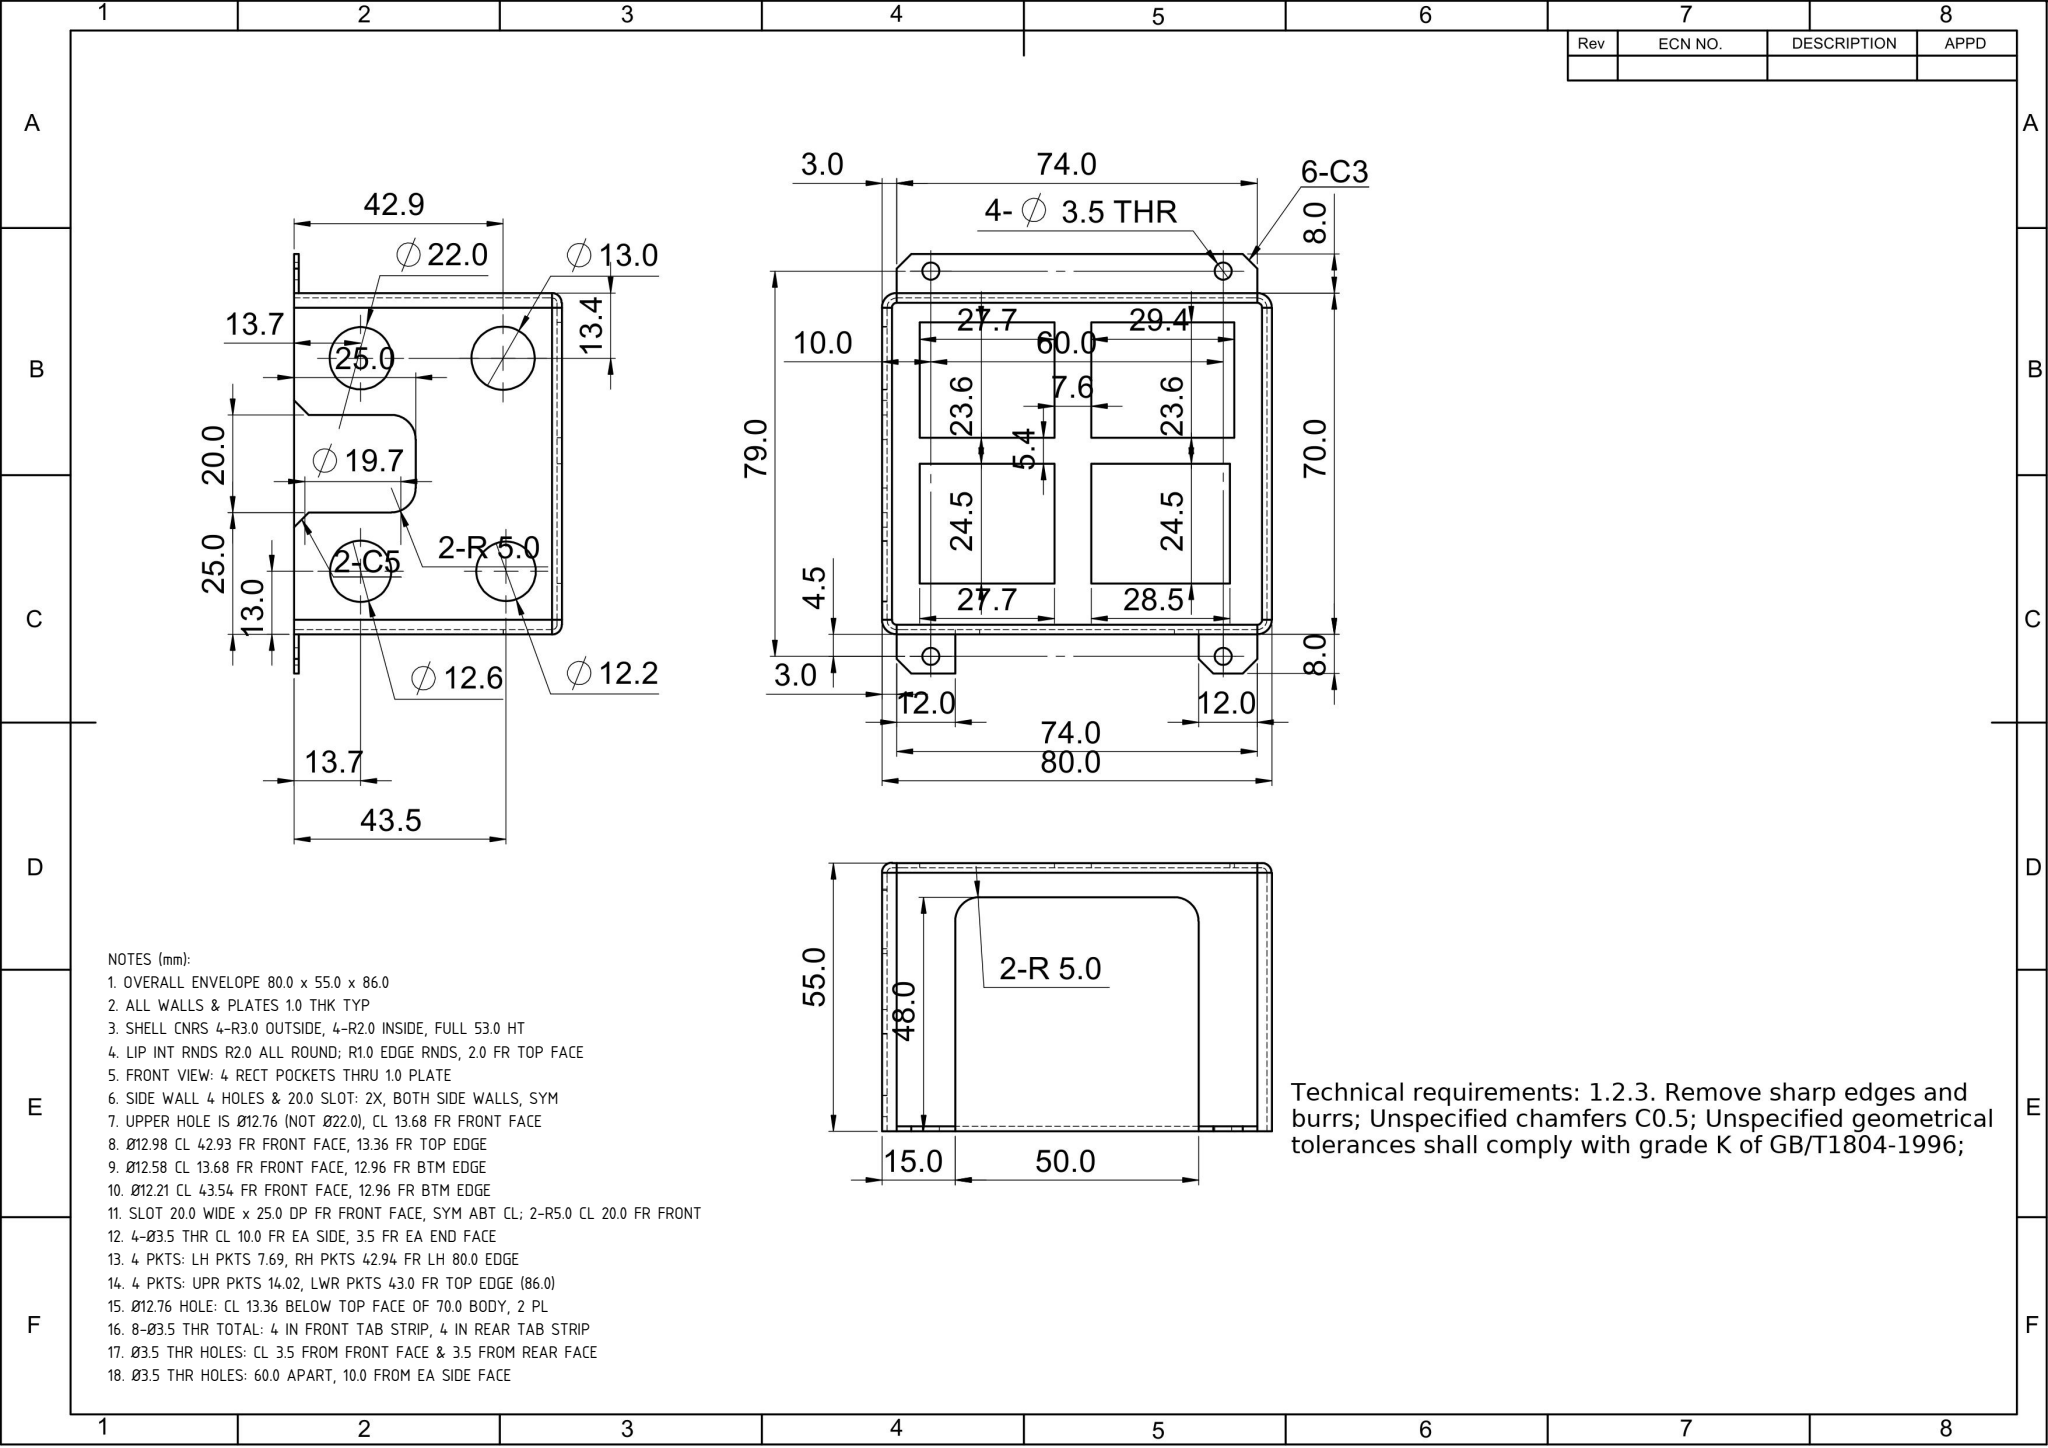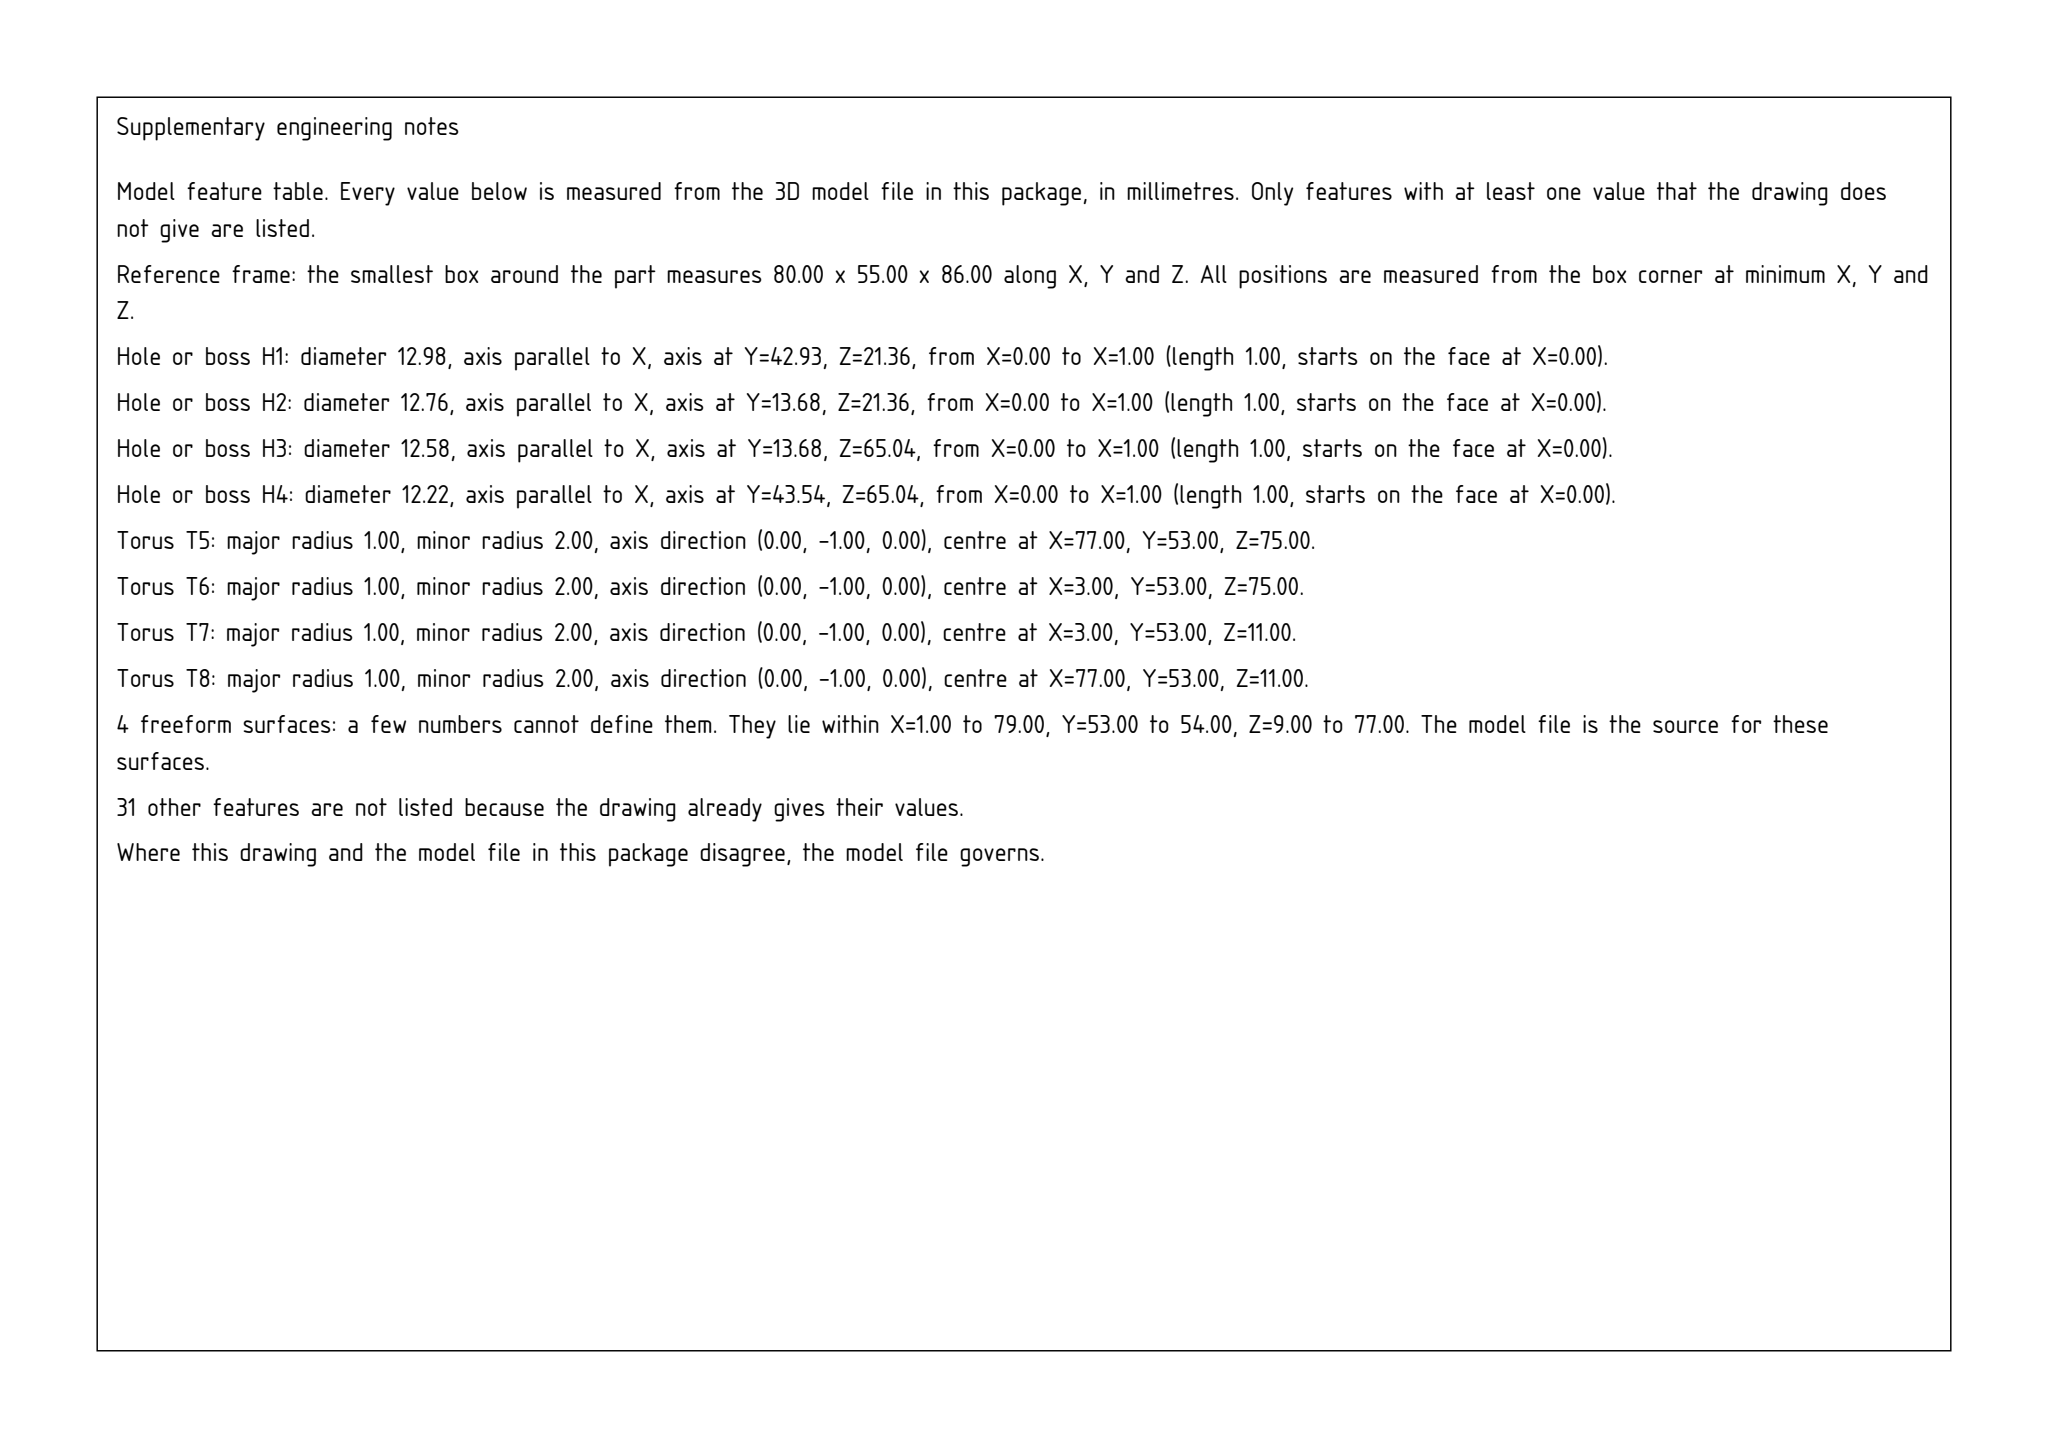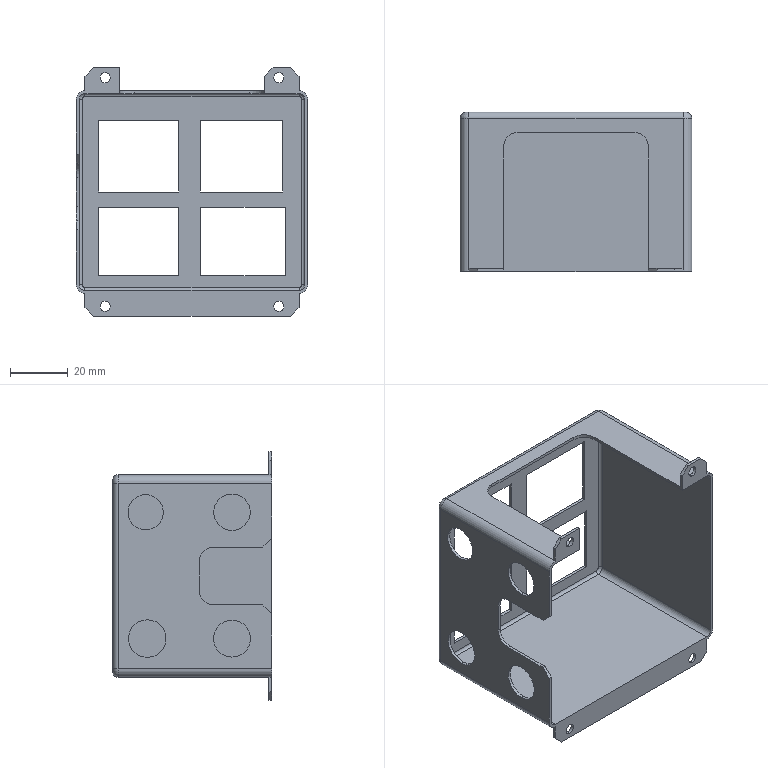Part | SolidWorks | mm | 1 solid | 95 faces | box 80 x 55 x 86 mm | volume 15740 mm3 | plane 51 | cylinder 36 | torus 4 | spline 4 | commonest cylinder face diameters 3.5 x8 4 x8 6 x4 10 x4 2 x4 12.213 x2 12.76 x2 12.582 x2
Drawing notes:
OVERALL ENVELOPE 80.0 x 55.0 x 86.0 | from the solid: bbox_xyz 80.0, 55.0, 86.0
ALL WALLS & PLATES 1.0 THK TYP | from the solid: Plane pairs x=0/1 & 79/80, y=0/1 & 54/55, z=8/9 & 77/78 all 1.0 apart
SHELL CNRS 4-R3.0 OUTSIDE, 4-R2.0 INSIDE, FULL 53.0 HT | from the solid: Ø6.0 y-axis cyls x4 at (3,11),(3,75),(77,11),(77,75) L=53 + Ø4.0 same pos = R3 out/R2 in
LIP INT RNDS R2.0 ALL ROUND; R1.0 EDGE RNDS, 2.0 FR TOP FACE | from the solid: Ø4.0 x- & z-axis cyls at y=53 (R2) and Ø2.0 x- & z-axis cyls at y=53 (R1); top face y=55
FRONT VIEW: 4 RECT POCKETS THRU 1.0 PLATE | from the solid: Only y-planes 0.0 and 1.0 bound pocketed face; no intermediate floor plane -> break thru
SIDE WALL 4 HOLES & 20.0 SLOT: 2X, BOTH SIDE WALLS, SYM | from the solid: count=2 for Ø12.213, Ø12.582, Ø12.76, Ø12.982 x-axis cyls; x-planes 0/1 and 79/80 walls
UPPER HOLE IS Ø12.76 (NOT Ø22.0), CL 13.68 FR FRONT FACE | from the solid: cyl Ø12.76 x-axis at y=13.68, z=21.36, L=1.0
Ø12.98 CL 42.93 FR FRONT FACE, 13.36 FR TOP EDGE | from the solid: cyl dia 12.982 axis x at (y=42.93, z=21.36); body edge z=8 -> 21.36-8=13.36
Ø12.58 CL 13.68 FR FRONT FACE, 12.96 FR BTM EDGE | from the solid: cyl dia 12.582 axis x at (y=13.68, z=65.04); body edge z=78 -> 78-65.04=12.96
Ø12.21 CL 43.54 FR FRONT FACE, 12.96 FR BTM EDGE | from the solid: cyl dia 12.213 axis x at (y=43.54, z=65.04); 78-65.04=12.96
SLOT 20.0 WIDE x 25.0 DP FR FRONT FACE, SYM ABT CL; 2-R5.0 CL 20.0 FR FRONT | from the solid: z-planes 33 & 53 (20.0 wide, CL z=43), ends y=25.0; Ø10 x-axis cyls at y=20, z=38 & 48
4-Ø3.5 THR CL 10.0 FR EA SIDE, 3.5 FR EA END FACE | from the solid: Ø3.5 y-axis holes at x=10/70, z=3.5/82.5, L=1.0; bbox x=80, z=86
4 PKTS: LH PKTS 7.69, RH PKTS 42.94 FR LH 80.0 EDGE | from the solid: x planes 7.69 (pkt LH edge, 2 PL) and 42.94 (RH pkt LH edge, 2 PL) vs bbox x=0; widths 35.37-7.69=27.7, 72.31-42.94=29.4, 71.39-42.94=28.5
4 PKTS: UPR PKTS 14.02, LWR PKTS 43.0 FR TOP EDGE (86.0) | from the solid: z planes 14.02 & 43.0 (pkt upper edges) vs bbox z=0 top edge; 37.65-14.02=23.6, 67.54-43.0=24.5, gap 43.0-37.65=5.4
Ø12.76 HOLE: CL 13.36 BELOW TOP FACE OF 70.0 BODY, 2 PL | from the solid: cyl dia 12.76 axis x at y=13.68, z=21.36, len 1.0, count 2; body top face z plane = 8.0, 21.36-8.0=13.36
8-Ø3.5 THR TOTAL: 4 IN FRONT TAB STRIP, 4 IN REAR TAB STRIP | from the solid: 3.5 dia cyl, axis y, at (x=10,z=3.5),(10,82.5),(70,3.5),(70,82.5), 2 each = 8
Ø3.5 THR HOLES: CL 3.5 FROM FRONT FACE & 3.5 FROM REAR FACE | from the solid: z=3.5 and z=82.5 with bbox z 0 to 86.0 (86-82.5=3.5)
Ø3.5 THR HOLES: 60.0 APART, 10.0 FROM EA SIDE FACE | from the solid: x=10.0 and x=70.0, bbox x 0 to 80.0